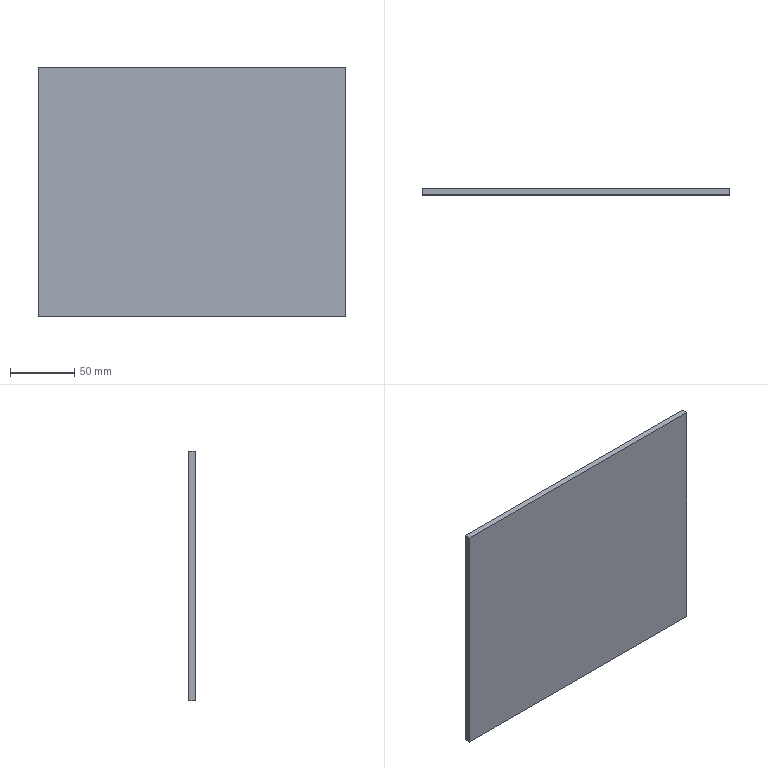Component | SolidWorks | 002FrameBaseAssembly-1_002FrameBasePanel2-1 | 1 solid | 6 faces | box 240 x 5 x 195 mm | volume 234000 mm3 | plane 6 | material Plain Carbon Steel
build123d program:
from build123d import *

# Parameters (mm, degrees)
SKETCH1_W           = 195
SKETCH1_H           = 240
BOSS_EXTRUDE1_DEPTH = 5


with BuildPart() as part:
    # Sketch1 → Boss-Extrude1 (new body)
    with BuildSketch(Plane.XY):
        Rectangle(SKETCH1_W, SKETCH1_H)
    extrude(amount=BOSS_EXTRUDE1_DEPTH)


solid = part.part

# Placed as in the assembly
solid = solid.moved(Location((260, 37, -262.5), (90, 0, 90)))
STEP:
#1=COLOUR_RGB('',0.7922,0.8196,0.9333);
#2=FILL_AREA_STYLE_COLOUR('',#1);
#3=FILL_AREA_STYLE('',(#2));
#4=SURFACE_STYLE_FILL_AREA(#3);
#5=SURFACE_SIDE_STYLE('',(#4));
#6=SURFACE_STYLE_USAGE(.BOTH.,#5);
#7=PRESENTATION_STYLE_ASSIGNMENT((#6));
#8=CARTESIAN_POINT('',(5.512,1.457,-14.173));
#9=VERTEX_POINT('',#8);
#10=CARTESIAN_POINT('',(14.961,1.457,-14.173));
#11=VERTEX_POINT('',#10);
#12=CARTESIAN_POINT('',(14.961,1.457,-14.173));
#13=DIRECTION('',(1.,-0.,0.));
#14=VECTOR('',#13,39.37);
#15=LINE('',#12,#14);
#16=EDGE_CURVE('',#9,#11,#15,.T.);
#17=ORIENTED_EDGE('',*,*,#16,.T.);
#18=CARTESIAN_POINT('',(14.961,1.26,-14.173));
#19=VERTEX_POINT('',#18);
#20=CARTESIAN_POINT('',(14.961,1.26,-14.173));
#21=DIRECTION('',(0.,1.,-0.));
#22=VECTOR('',#21,39.37);
#23=LINE('',#20,#22);
#24=EDGE_CURVE('',#19,#11,#23,.T.);
#25=ORIENTED_EDGE('',*,*,#24,.F.);
#26=CARTESIAN_POINT('',(5.512,1.26,-14.173));
#27=VERTEX_POINT('',#26);
#28=CARTESIAN_POINT('',(14.961,1.26,-14.173));
#29=DIRECTION('',(1.,-0.,0.));
#30=VECTOR('',#29,39.37);
#31=LINE('',#28,#30);
#32=EDGE_CURVE('',#27,#19,#31,.T.);
#33=ORIENTED_EDGE('',*,*,#32,.F.);
#34=CARTESIAN_POINT('',(5.512,1.26,-14.173));
#35=DIRECTION('',(0.,1.,-0.));
#36=VECTOR('',#35,39.37);
#37=LINE('',#34,#36);
#38=EDGE_CURVE('',#27,#9,#37,.T.);
#39=ORIENTED_EDGE('',*,*,#38,.T.);
#40=EDGE_LOOP('',(#17,#25,#33,#39));
#41=FACE_OUTER_BOUND('',#40,.T.);
#42=CARTESIAN_POINT('',(14.961,1.26,-14.173));
#43=DIRECTION('',(-0.,0.,1.));
#44=DIRECTION('',(-1.,0.,-0.));
#45=AXIS2_PLACEMENT_3D('',#42,#43,#44);
#46=PLANE('',#45);
#47=ADVANCED_FACE('',(#41),#46,.F.);
#48=CARTESIAN_POINT('',(14.961,1.457,-6.496));
#49=VERTEX_POINT('',#48);
#50=CARTESIAN_POINT('',(14.961,1.457,-6.496));
#51=DIRECTION('',(0.,0.,1.));
#52=VECTOR('',#51,39.37);
#53=LINE('',#50,#52);
#54=EDGE_CURVE('',#11,#49,#53,.T.);
#55=ORIENTED_EDGE('',*,*,#54,.T.);
#56=CARTESIAN_POINT('',(14.961,1.26,-6.496));
#57=VERTEX_POINT('',#56);
#58=CARTESIAN_POINT('',(14.961,1.26,-6.496));
#59=DIRECTION('',(0.,1.,-0.));
#60=VECTOR('',#59,39.37);
#61=LINE('',#58,#60);
#62=EDGE_CURVE('',#57,#49,#61,.T.);
#63=ORIENTED_EDGE('',*,*,#62,.F.);
#64=CARTESIAN_POINT('',(14.961,1.26,-6.496));
#65=DIRECTION('',(0.,0.,1.));
#66=VECTOR('',#65,39.37);
#67=LINE('',#64,#66);
#68=EDGE_CURVE('',#19,#57,#67,.T.);
#69=ORIENTED_EDGE('',*,*,#68,.F.);
#70=ORIENTED_EDGE('',*,*,#24,.T.);
#71=EDGE_LOOP('',(#55,#63,#69,#70));
#72=FACE_OUTER_BOUND('',#71,.T.);
#73=CARTESIAN_POINT('',(14.961,1.26,-6.496));
#74=DIRECTION('',(-1.,0.,0.));
#75=DIRECTION('',(0.,1.,-0.));
#76=AXIS2_PLACEMENT_3D('',#73,#74,#75);
#77=PLANE('',#76);
#78=ADVANCED_FACE('',(#72),#77,.F.);
#79=CARTESIAN_POINT('',(5.512,1.457,-6.496));
#80=VERTEX_POINT('',#79);
#81=CARTESIAN_POINT('',(14.961,1.457,-6.496));
#82=DIRECTION('',(-1.,0.,-0.));
#83=VECTOR('',#82,39.37);
#84=LINE('',#81,#83);
#85=EDGE_CURVE('',#49,#80,#84,.T.);
#86=ORIENTED_EDGE('',*,*,#85,.T.);
#87=CARTESIAN_POINT('',(5.512,1.26,-6.496));
#88=VERTEX_POINT('',#87);
#89=CARTESIAN_POINT('',(5.512,1.26,-6.496));
#90=DIRECTION('',(0.,1.,-0.));
#91=VECTOR('',#90,39.37);
#92=LINE('',#89,#91);
#93=EDGE_CURVE('',#88,#80,#92,.T.);
#94=ORIENTED_EDGE('',*,*,#93,.F.);
#95=CARTESIAN_POINT('',(14.961,1.26,-6.496));
#96=DIRECTION('',(-1.,0.,-0.));
#97=VECTOR('',#96,39.37);
#98=LINE('',#95,#97);
#99=EDGE_CURVE('',#57,#88,#98,.T.);
#100=ORIENTED_EDGE('',*,*,#99,.F.);
#101=ORIENTED_EDGE('',*,*,#62,.T.);
#102=EDGE_LOOP('',(#86,#94,#100,#101));
#103=FACE_OUTER_BOUND('',#102,.T.);
#104=CARTESIAN_POINT('',(14.961,1.26,-6.496));
#105=DIRECTION('',(0.,-0.,-1.));
#106=DIRECTION('',(1.,-0.,0.));
#107=AXIS2_PLACEMENT_3D('',#104,#105,#106);
#108=PLANE('',#107);
#109=ADVANCED_FACE('',(#103),#108,.F.);
#110=CARTESIAN_POINT('',(5.512,1.457,-6.496));
#111=DIRECTION('',(-0.,-0.,-1.));
#112=VECTOR('',#111,39.37);
#113=LINE('',#110,#112);
#114=EDGE_CURVE('',#80,#9,#113,.T.);
#115=ORIENTED_EDGE('',*,*,#114,.T.);
#116=ORIENTED_EDGE('',*,*,#38,.F.);
#117=CARTESIAN_POINT('',(5.512,1.26,-6.496));
#118=DIRECTION('',(-0.,-0.,-1.));
#119=VECTOR('',#118,39.37);
#120=LINE('',#117,#119);
#121=EDGE_CURVE('',#88,#27,#120,.T.);
#122=ORIENTED_EDGE('',*,*,#121,.F.);
#123=ORIENTED_EDGE('',*,*,#93,.T.);
#124=EDGE_LOOP('',(#115,#116,#122,#123));
#125=FACE_OUTER_BOUND('',#124,.T.);
#126=CARTESIAN_POINT('',(5.512,1.26,-6.496));
#127=DIRECTION('',(1.,-0.,0.));
#128=DIRECTION('',(-0.,-1.,0.));
#129=AXIS2_PLACEMENT_3D('',#126,#127,#128);
#130=PLANE('',#129);
#131=ADVANCED_FACE('',(#125),#130,.F.);
#132=ORIENTED_EDGE('',*,*,#32,.T.);
#133=ORIENTED_EDGE('',*,*,#68,.T.);
#134=ORIENTED_EDGE('',*,*,#99,.T.);
#135=ORIENTED_EDGE('',*,*,#121,.T.);
#136=EDGE_LOOP('',(#132,#133,#134,#135));
#137=FACE_OUTER_BOUND('',#136,.T.);
#138=CARTESIAN_POINT('',(5.512,1.26,-14.173));
#139=DIRECTION('',(-0.,-1.,0.));
#140=DIRECTION('',(-0.,-0.,-1.));
#141=AXIS2_PLACEMENT_3D('',#138,#139,#140);
#142=PLANE('',#141);
#143=ADVANCED_FACE('',(#137),#142,.T.);
#144=ORIENTED_EDGE('',*,*,#16,.F.);
#145=ORIENTED_EDGE('',*,*,#114,.F.);
#146=ORIENTED_EDGE('',*,*,#85,.F.);
#147=ORIENTED_EDGE('',*,*,#54,.F.);
#148=EDGE_LOOP('',(#144,#145,#146,#147));
#149=FACE_OUTER_BOUND('',#148,.T.);
#150=CARTESIAN_POINT('',(5.512,1.457,-14.173));
#151=DIRECTION('',(-0.,-1.,0.));
#152=DIRECTION('',(-0.,-0.,-1.));
#153=AXIS2_PLACEMENT_3D('',#150,#151,#152);
#154=PLANE('',#153);
#155=ADVANCED_FACE('',(#149),#154,.F.);
#156=CLOSED_SHELL('',(#47,#78,#109,#131,#143,#155));
#157=MANIFOLD_SOLID_BREP('',#156);
#158=STYLED_ITEM('',(#7),#157);
#159=PRESENTATION_LAYER_ASSIGNMENT('','',(#158));
#160=CARTESIAN_POINT('',(0.,0.,0.));
#161=DIRECTION('',(0.,0.,1.));
#162=DIRECTION('',(1.,0.,0.));
#163=AXIS2_PLACEMENT_3D('',#160,#161,#162);
#164=(LENGTH_UNIT()NAMED_UNIT(*)SI_UNIT($,.METRE.));
#165=LENGTH_MEASURE_WITH_UNIT(LENGTH_MEASURE(0.0254),#164);
#166=DIMENSIONAL_EXPONENTS(1.,0.,0.,0.,0.,0.,0.);
#167=(CONVERSION_BASED_UNIT('',#165)LENGTH_UNIT()NAMED_UNIT(#166));
#168=UNCERTAINTY_MEASURE_WITH_UNIT(LENGTH_MEASURE(0.00001),#167,'','');
#169=(NAMED_UNIT(*)PLANE_ANGLE_UNIT()SI_UNIT($,.RADIAN.));
#170=(NAMED_UNIT(*)SI_UNIT($,.STERADIAN.)SOLID_ANGLE_UNIT());
#171=(GEOMETRIC_REPRESENTATION_CONTEXT(3)GLOBAL_UNCERTAINTY_ASSIGNED_CONTEXT((#168))GLOBAL_UNIT_ASSIGNED_CONTEXT((#167,#169,#170))REPRESENTATION_CONTEXT('',''));
#172=ADVANCED_BREP_SHAPE_REPRESENTATION('',(#157,#163),#171);
#173=(LENGTH_UNIT()NAMED_UNIT(*)SI_UNIT($,.METRE.));
#174=LENGTH_MEASURE_WITH_UNIT(LENGTH_MEASURE(0.0254),#173);
#175=DIMENSIONAL_EXPONENTS(1.,0.,0.,0.,0.,0.,0.);
#176=(CONVERSION_BASED_UNIT('',#174)LENGTH_UNIT()NAMED_UNIT(#175));
#177=UNCERTAINTY_MEASURE_WITH_UNIT(LENGTH_MEASURE(0.00001),#176,'','');
#178=(NAMED_UNIT(*)PLANE_ANGLE_UNIT()SI_UNIT($,.RADIAN.));
#179=(NAMED_UNIT(*)SI_UNIT($,.STERADIAN.)SOLID_ANGLE_UNIT());
#180=(GEOMETRIC_REPRESENTATION_CONTEXT(3)GLOBAL_UNCERTAINTY_ASSIGNED_CONTEXT((#177))GLOBAL_UNIT_ASSIGNED_CONTEXT((#176,#178,#179))REPRESENTATION_CONTEXT('',''));
#181=MECHANICAL_DESIGN_GEOMETRIC_PRESENTATION_REPRESENTATION('',(#158),#180);